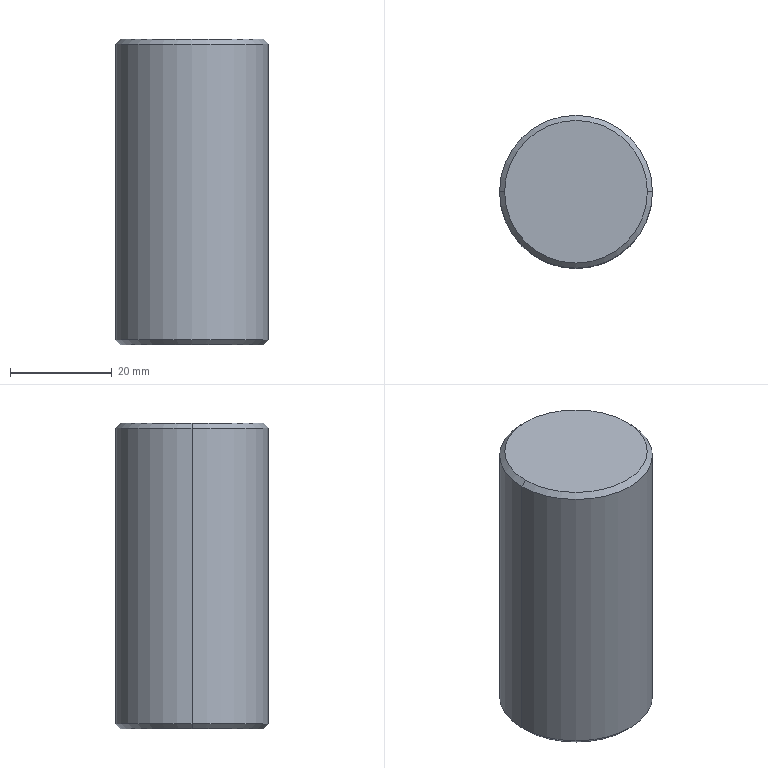Component | SolidWorks | CenterAxis-1 | 1 solid | 8 faces | box 30 x 30 x 60 mm | volume 42319 mm3 | cone 4 | cylinder 2 | plane 2 | commonest cylinder face diameters 30 x2
build123d program:
from build123d import *

# Parameters (mm, degrees)
SKETCH1_R           = 15
BOSS_EXTRUDE1_DEPTH = 60
CHAMFER1_SIZE       = 1


with BuildPart() as part:
    # Sketch1 → Boss-Extrude1 (new body)
    with BuildSketch(Plane.XY):
        Circle(SKETCH1_R)
    extrude(amount=BOSS_EXTRUDE1_DEPTH)

    # Chamfer1
    chamfer1_edges = [part.edges().sort_by_distance(p)[0] for p in [
        (-15, 0, 0),
        (-15, 0, 60),
    ]]
    chamfer(chamfer1_edges, length=CHAMFER1_SIZE)


solid = part.part

# Placed as in the assembly
solid = solid.moved(Location((61.422, 112.819, 13.038), (0, 0, 0)))
STEP:
#1=CARTESIAN_POINT('',(1.867,4.442,0.5133));
#2=VERTEX_POINT('',#1);
#3=CARTESIAN_POINT('',(2.969,4.442,0.5133));
#4=VERTEX_POINT('',#3);
#5=CARTESIAN_POINT('',(2.418,4.442,0.5133));
#6=DIRECTION('',(0.,0.,-1.));
#7=DIRECTION('',(1.,0.,0.));
#8=AXIS2_PLACEMENT_3D('',#5,#6,#7);
#9=CIRCLE('',#8,0.5512);
#10=EDGE_CURVE('',#2,#4,#9,.T.);
#11=ORIENTED_EDGE('',*,*,#10,.F.);
#12=CARTESIAN_POINT('',(1.828,4.442,0.5527));
#13=VERTEX_POINT('',#12);
#14=CARTESIAN_POINT('',(1.828,4.442,0.5527));
#15=DIRECTION('',(-0.7071,0.,0.7071));
#16=VECTOR('',#15,39.37);
#17=LINE('',#14,#16);
#18=EDGE_CURVE('',#2,#13,#17,.T.);
#19=ORIENTED_EDGE('',*,*,#18,.T.);
#20=CARTESIAN_POINT('',(3.009,4.442,0.5527));
#21=VERTEX_POINT('',#20);
#22=CARTESIAN_POINT('',(2.418,4.442,0.5527));
#23=DIRECTION('',(0.,0.,1.));
#24=DIRECTION('',(1.,0.,0.));
#25=AXIS2_PLACEMENT_3D('',#22,#23,#24);
#26=CIRCLE('',#25,0.5906);
#27=EDGE_CURVE('',#21,#13,#26,.T.);
#28=ORIENTED_EDGE('',*,*,#27,.F.);
#29=CARTESIAN_POINT('',(3.009,4.442,0.5527));
#30=DIRECTION('',(0.7071,0.,0.7071));
#31=VECTOR('',#30,39.37);
#32=LINE('',#29,#31);
#33=EDGE_CURVE('',#4,#21,#32,.T.);
#34=ORIENTED_EDGE('',*,*,#33,.F.);
#35=EDGE_LOOP('',(#11,#19,#28,#34));
#36=FACE_OUTER_BOUND('',#35,.T.);
#37=CARTESIAN_POINT('',(2.418,4.442,0.5527));
#38=DIRECTION('',(0.,0.,1.));
#39=DIRECTION('',(1.,0.,0.));
#40=AXIS2_PLACEMENT_3D('',#37,#38,#39);
#41=CONICAL_SURFACE('',#40,0.5906,0.7854);
#42=ADVANCED_FACE('',(#36),#41,.T.);
#43=CARTESIAN_POINT('',(2.969,4.442,2.875));
#44=VERTEX_POINT('',#43);
#45=CARTESIAN_POINT('',(1.867,4.442,2.875));
#46=VERTEX_POINT('',#45);
#47=CARTESIAN_POINT('',(2.418,4.442,2.875));
#48=DIRECTION('',(0.,0.,1.));
#49=DIRECTION('',(1.,0.,0.));
#50=AXIS2_PLACEMENT_3D('',#47,#48,#49);
#51=CIRCLE('',#50,0.5512);
#52=EDGE_CURVE('',#44,#46,#51,.T.);
#53=ORIENTED_EDGE('',*,*,#52,.F.);
#54=CARTESIAN_POINT('',(3.009,4.442,2.836));
#55=VERTEX_POINT('',#54);
#56=CARTESIAN_POINT('',(2.969,4.442,2.875));
#57=DIRECTION('',(0.7071,0.,-0.7071));
#58=VECTOR('',#57,39.37);
#59=LINE('',#56,#58);
#60=EDGE_CURVE('',#44,#55,#59,.T.);
#61=ORIENTED_EDGE('',*,*,#60,.T.);
#62=CARTESIAN_POINT('',(1.828,4.442,2.836));
#63=VERTEX_POINT('',#62);
#64=CARTESIAN_POINT('',(2.418,4.442,2.836));
#65=DIRECTION('',(0.,0.,-1.));
#66=DIRECTION('',(1.,0.,0.));
#67=AXIS2_PLACEMENT_3D('',#64,#65,#66);
#68=CIRCLE('',#67,0.5906);
#69=EDGE_CURVE('',#63,#55,#68,.T.);
#70=ORIENTED_EDGE('',*,*,#69,.F.);
#71=CARTESIAN_POINT('',(1.867,4.442,2.875));
#72=DIRECTION('',(-0.7071,0.,-0.7071));
#73=VECTOR('',#72,39.37);
#74=LINE('',#71,#73);
#75=EDGE_CURVE('',#46,#63,#74,.T.);
#76=ORIENTED_EDGE('',*,*,#75,.F.);
#77=EDGE_LOOP('',(#53,#61,#70,#76));
#78=FACE_OUTER_BOUND('',#77,.T.);
#79=CARTESIAN_POINT('',(2.418,4.442,2.875));
#80=DIRECTION('',(0.,0.,-1.));
#81=DIRECTION('',(-1.,0.,0.));
#82=AXIS2_PLACEMENT_3D('',#79,#80,#81);
#83=CONICAL_SURFACE('',#82,0.5512,0.7854);
#84=ADVANCED_FACE('',(#78),#83,.T.);
#85=ORIENTED_EDGE('',*,*,#69,.T.);
#86=CARTESIAN_POINT('',(3.009,4.442,2.875));
#87=DIRECTION('',(0.,0.,-1.));
#88=VECTOR('',#87,39.37);
#89=LINE('',#86,#88);
#90=EDGE_CURVE('',#55,#21,#89,.T.);
#91=ORIENTED_EDGE('',*,*,#90,.T.);
#92=ORIENTED_EDGE('',*,*,#27,.T.);
#93=CARTESIAN_POINT('',(1.828,4.442,2.875));
#94=DIRECTION('',(0.,0.,-1.));
#95=VECTOR('',#94,39.37);
#96=LINE('',#93,#95);
#97=EDGE_CURVE('',#63,#13,#96,.T.);
#98=ORIENTED_EDGE('',*,*,#97,.F.);
#99=EDGE_LOOP('',(#85,#91,#92,#98));
#100=FACE_OUTER_BOUND('',#99,.T.);
#101=CARTESIAN_POINT('',(2.418,4.442,2.875));
#102=DIRECTION('',(0.,0.,-1.));
#103=DIRECTION('',(-1.,0.,0.));
#104=AXIS2_PLACEMENT_3D('',#101,#102,#103);
#105=CYLINDRICAL_SURFACE('',#104,0.5906);
#106=ADVANCED_FACE('',(#100),#105,.T.);
#107=ORIENTED_EDGE('',*,*,#90,.F.);
#108=CARTESIAN_POINT('',(2.418,4.442,2.836));
#109=DIRECTION('',(0.,0.,-1.));
#110=DIRECTION('',(1.,0.,0.));
#111=AXIS2_PLACEMENT_3D('',#108,#109,#110);
#112=CIRCLE('',#111,0.5906);
#113=EDGE_CURVE('',#55,#63,#112,.T.);
#114=ORIENTED_EDGE('',*,*,#113,.T.);
#115=ORIENTED_EDGE('',*,*,#97,.T.);
#116=CARTESIAN_POINT('',(2.418,4.442,0.5527));
#117=DIRECTION('',(0.,0.,1.));
#118=DIRECTION('',(1.,0.,0.));
#119=AXIS2_PLACEMENT_3D('',#116,#117,#118);
#120=CIRCLE('',#119,0.5906);
#121=EDGE_CURVE('',#13,#21,#120,.T.);
#122=ORIENTED_EDGE('',*,*,#121,.T.);
#123=EDGE_LOOP('',(#107,#114,#115,#122));
#124=FACE_OUTER_BOUND('',#123,.T.);
#125=CARTESIAN_POINT('',(2.418,4.442,2.875));
#126=DIRECTION('',(0.,0.,-1.));
#127=DIRECTION('',(-1.,0.,0.));
#128=AXIS2_PLACEMENT_3D('',#125,#126,#127);
#129=CYLINDRICAL_SURFACE('',#128,0.5906);
#130=ADVANCED_FACE('',(#124),#129,.T.);
#131=CARTESIAN_POINT('',(2.418,4.442,2.875));
#132=DIRECTION('',(0.,0.,1.));
#133=DIRECTION('',(1.,0.,0.));
#134=AXIS2_PLACEMENT_3D('',#131,#132,#133);
#135=CIRCLE('',#134,0.5512);
#136=EDGE_CURVE('',#46,#44,#135,.T.);
#137=ORIENTED_EDGE('',*,*,#136,.T.);
#138=ORIENTED_EDGE('',*,*,#52,.T.);
#139=EDGE_LOOP('',(#137,#138));
#140=FACE_OUTER_BOUND('',#139,.T.);
#141=CARTESIAN_POINT('',(2.418,4.442,2.875));
#142=DIRECTION('',(0.,0.,1.));
#143=DIRECTION('',(1.,0.,0.));
#144=AXIS2_PLACEMENT_3D('',#141,#142,#143);
#145=PLANE('',#144);
#146=ADVANCED_FACE('',(#140),#145,.T.);
#147=CARTESIAN_POINT('',(2.418,4.442,0.5133));
#148=DIRECTION('',(0.,0.,-1.));
#149=DIRECTION('',(1.,0.,0.));
#150=AXIS2_PLACEMENT_3D('',#147,#148,#149);
#151=CIRCLE('',#150,0.5512);
#152=EDGE_CURVE('',#4,#2,#151,.T.);
#153=ORIENTED_EDGE('',*,*,#152,.T.);
#154=ORIENTED_EDGE('',*,*,#10,.T.);
#155=EDGE_LOOP('',(#153,#154));
#156=FACE_OUTER_BOUND('',#155,.T.);
#157=CARTESIAN_POINT('',(2.418,4.442,0.5133));
#158=DIRECTION('',(0.,0.,1.));
#159=DIRECTION('',(1.,0.,0.));
#160=AXIS2_PLACEMENT_3D('',#157,#158,#159);
#161=PLANE('',#160);
#162=ADVANCED_FACE('',(#156),#161,.F.);
#163=ORIENTED_EDGE('',*,*,#60,.F.);
#164=ORIENTED_EDGE('',*,*,#136,.F.);
#165=ORIENTED_EDGE('',*,*,#75,.T.);
#166=ORIENTED_EDGE('',*,*,#113,.F.);
#167=EDGE_LOOP('',(#163,#164,#165,#166));
#168=FACE_OUTER_BOUND('',#167,.T.);
#169=CARTESIAN_POINT('',(2.418,4.442,2.875));
#170=DIRECTION('',(0.,0.,-1.));
#171=DIRECTION('',(-1.,0.,0.));
#172=AXIS2_PLACEMENT_3D('',#169,#170,#171);
#173=CONICAL_SURFACE('',#172,0.5512,0.7854);
#174=ADVANCED_FACE('',(#168),#173,.T.);
#175=ORIENTED_EDGE('',*,*,#18,.F.);
#176=ORIENTED_EDGE('',*,*,#152,.F.);
#177=ORIENTED_EDGE('',*,*,#33,.T.);
#178=ORIENTED_EDGE('',*,*,#121,.F.);
#179=EDGE_LOOP('',(#175,#176,#177,#178));
#180=FACE_OUTER_BOUND('',#179,.T.);
#181=CARTESIAN_POINT('',(2.418,4.442,0.5527));
#182=DIRECTION('',(0.,0.,1.));
#183=DIRECTION('',(1.,0.,0.));
#184=AXIS2_PLACEMENT_3D('',#181,#182,#183);
#185=CONICAL_SURFACE('',#184,0.5906,0.7854);
#186=ADVANCED_FACE('',(#180),#185,.T.);
#187=CLOSED_SHELL('',(#42,#84,#106,#130,#146,#162,#174,#186));
#188=MANIFOLD_SOLID_BREP('',#187);
#189=CARTESIAN_POINT('',(0.,0.,0.));
#190=DIRECTION('',(0.,0.,1.));
#191=DIRECTION('',(1.,0.,0.));
#192=AXIS2_PLACEMENT_3D('',#189,#190,#191);
#193=(LENGTH_UNIT()NAMED_UNIT(*)SI_UNIT($,.METRE.));
#194=LENGTH_MEASURE_WITH_UNIT(LENGTH_MEASURE(0.0254),#193);
#195=DIMENSIONAL_EXPONENTS(1.,0.,0.,0.,0.,0.,0.);
#196=(CONVERSION_BASED_UNIT('',#194)LENGTH_UNIT()NAMED_UNIT(#195));
#197=UNCERTAINTY_MEASURE_WITH_UNIT(LENGTH_MEASURE(0.00001),#196,'','');
#198=(NAMED_UNIT(*)PLANE_ANGLE_UNIT()SI_UNIT($,.RADIAN.));
#199=(NAMED_UNIT(*)SI_UNIT($,.STERADIAN.)SOLID_ANGLE_UNIT());
#200=(GEOMETRIC_REPRESENTATION_CONTEXT(3)GLOBAL_UNCERTAINTY_ASSIGNED_CONTEXT((#197))GLOBAL_UNIT_ASSIGNED_CONTEXT((#196,#198,#199))REPRESENTATION_CONTEXT('',''));
#201=ADVANCED_BREP_SHAPE_REPRESENTATION('',(#188,#192),#200);
#202=COLOUR_RGB('',0.7922,0.8196,0.9333);
#203=FILL_AREA_STYLE_COLOUR('',#202);
#204=FILL_AREA_STYLE('',(#203));
#205=SURFACE_STYLE_FILL_AREA(#204);
#206=SURFACE_SIDE_STYLE('',(#205));
#207=SURFACE_STYLE_USAGE(.BOTH.,#206);
#208=PRESENTATION_STYLE_ASSIGNMENT((#207));
#209=STYLED_ITEM('',(#208),#188);
#210=(LENGTH_UNIT()NAMED_UNIT(*)SI_UNIT($,.METRE.));
#211=LENGTH_MEASURE_WITH_UNIT(LENGTH_MEASURE(0.0254),#210);
#212=DIMENSIONAL_EXPONENTS(1.,0.,0.,0.,0.,0.,0.);
#213=(CONVERSION_BASED_UNIT('',#211)LENGTH_UNIT()NAMED_UNIT(#212));
#214=UNCERTAINTY_MEASURE_WITH_UNIT(LENGTH_MEASURE(0.00001),#213,'','');
#215=(NAMED_UNIT(*)PLANE_ANGLE_UNIT()SI_UNIT($,.RADIAN.));
#216=(NAMED_UNIT(*)SI_UNIT($,.STERADIAN.)SOLID_ANGLE_UNIT());
#217=(GEOMETRIC_REPRESENTATION_CONTEXT(3)GLOBAL_UNCERTAINTY_ASSIGNED_CONTEXT((#214))GLOBAL_UNIT_ASSIGNED_CONTEXT((#213,#215,#216))REPRESENTATION_CONTEXT('',''));
#218=MECHANICAL_DESIGN_GEOMETRIC_PRESENTATION_REPRESENTATION('',(#209),#217);
#219=PRESENTATION_LAYER_ASSIGNMENT('','',(#209));